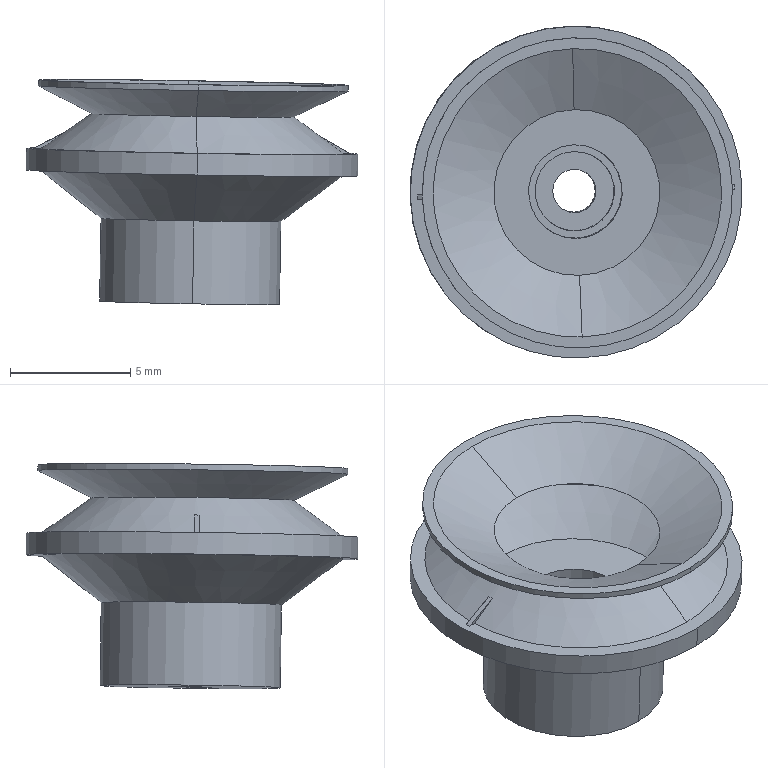Component | SolidWorks | 00-VacuumSuctionCupAssembly-1_08-SoftRubberSuctionCup-28 | 1 solid | 37 faces | box 13.81 x 13.81 x 9.37 mm | volume 326 mm3 | plane 13 | cylinder 12 | cone 12 | commonest cylinder face diameters 1.8 x2 3.9 x2 3.3 x2 7.5 x2 12.9 x2 13.8 x2
STEP:
#1=COLOUR_RGB('',0.7922,0.8196,0.9333);
#2=FILL_AREA_STYLE_COLOUR('',#1);
#3=FILL_AREA_STYLE('',(#2));
#4=SURFACE_STYLE_FILL_AREA(#3);
#5=SURFACE_SIDE_STYLE('',(#4));
#6=SURFACE_STYLE_USAGE(.BOTH.,#5);
#7=PRESENTATION_STYLE_ASSIGNMENT((#6));
#8=CARTESIAN_POINT('',(1.624,5.222,2.221));
#9=VERTEX_POINT('',#8);
#10=CARTESIAN_POINT('',(1.622,5.292,2.222));
#11=VERTEX_POINT('',#10);
#12=CARTESIAN_POINT('',(1.623,5.257,2.222));
#13=DIRECTION('',(0.01745,-0.01259,0.9998));
#14=DIRECTION('',(0.03309,-0.9994,-0.01316));
#15=AXIS2_PLACEMENT_3D('',#12,#13,#14);
#16=CIRCLE('',#15,0.03543);
#17=EDGE_CURVE('',#9,#11,#16,.T.);
#18=ORIENTED_EDGE('',*,*,#17,.F.);
#19=CARTESIAN_POINT('',(1.625,5.221,2.304));
#20=VERTEX_POINT('',#19);
#21=CARTESIAN_POINT('',(1.622,5.223,2.127));
#22=DIRECTION('',(0.01745,-0.01259,0.9998));
#23=VECTOR('',#22,39.37);
#24=LINE('',#21,#23);
#25=EDGE_CURVE('',#9,#20,#24,.T.);
#26=ORIENTED_EDGE('',*,*,#25,.T.);
#27=CARTESIAN_POINT('',(1.623,5.291,2.305));
#28=VERTEX_POINT('',#27);
#29=CARTESIAN_POINT('',(1.624,5.256,2.305));
#30=DIRECTION('',(-0.01745,0.01259,-0.9998));
#31=DIRECTION('',(0.03309,-0.9994,-0.01316));
#32=AXIS2_PLACEMENT_3D('',#29,#30,#31);
#33=CIRCLE('',#32,0.03543);
#34=EDGE_CURVE('',#28,#20,#33,.T.);
#35=ORIENTED_EDGE('',*,*,#34,.F.);
#36=CARTESIAN_POINT('',(1.62,5.294,2.128));
#37=DIRECTION('',(0.01745,-0.01259,0.9998));
#38=VECTOR('',#37,39.37);
#39=LINE('',#36,#38);
#40=EDGE_CURVE('',#11,#28,#39,.T.);
#41=ORIENTED_EDGE('',*,*,#40,.F.);
#42=EDGE_LOOP('',(#18,#26,#35,#41));
#43=FACE_OUTER_BOUND('',#42,.T.);
#44=CARTESIAN_POINT('',(1.621,5.258,2.127));
#45=DIRECTION('',(0.01745,-0.01259,0.9998));
#46=DIRECTION('',(-0.03309,0.9994,0.01316));
#47=AXIS2_PLACEMENT_3D('',#44,#45,#46);
#48=CYLINDRICAL_SURFACE('',#47,0.03543);
#49=ADVANCED_FACE('',(#43),#48,.F.);
#50=CARTESIAN_POINT('',(1.624,5.389,2.531));
#51=VERTEX_POINT('',#50);
#52=CARTESIAN_POINT('',(1.633,5.117,2.527));
#53=VERTEX_POINT('',#52);
#54=CARTESIAN_POINT('',(1.628,5.253,2.529));
#55=DIRECTION('',(-0.01745,0.01259,-0.9998));
#56=DIRECTION('',(0.03309,-0.9994,-0.01316));
#57=AXIS2_PLACEMENT_3D('',#54,#55,#56);
#58=CIRCLE('',#57,0.1358);
#59=EDGE_CURVE('',#51,#53,#58,.T.);
#60=ORIENTED_EDGE('',*,*,#59,.F.);
#61=CARTESIAN_POINT('',(1.619,5.492,2.459));
#62=VERTEX_POINT('',#61);
#63=CARTESIAN_POINT('',(1.619,5.492,2.459));
#64=DIRECTION('',(-0.03707,0.8205,-0.5704));
#65=VECTOR('',#64,39.37);
#66=LINE('',#63,#65);
#67=EDGE_CURVE('',#51,#62,#66,.T.);
#68=ORIENTED_EDGE('',*,*,#67,.T.);
#69=CARTESIAN_POINT('',(1.635,5.016,2.453));
#70=VERTEX_POINT('',#69);
#71=CARTESIAN_POINT('',(1.627,5.254,2.456));
#72=DIRECTION('',(-0.01745,0.01259,-0.9998));
#73=DIRECTION('',(0.03309,-0.9994,-0.01316));
#74=AXIS2_PLACEMENT_3D('',#71,#72,#73);
#75=CIRCLE('',#74,0.2381);
#76=EDGE_CURVE('',#62,#70,#75,.T.);
#77=ORIENTED_EDGE('',*,*,#76,.T.);
#78=CARTESIAN_POINT('',(1.635,5.016,2.453));
#79=DIRECTION('',(0.01679,-0.8059,-0.5918));
#80=VECTOR('',#79,39.37);
#81=LINE('',#78,#80);
#82=EDGE_CURVE('',#53,#70,#81,.T.);
#83=ORIENTED_EDGE('',*,*,#82,.F.);
#84=EDGE_LOOP('',(#60,#68,#77,#83));
#85=FACE_OUTER_BOUND('',#84,.T.);
#86=CARTESIAN_POINT('',(1.627,5.254,2.456));
#87=DIRECTION('',(-0.01745,0.01259,-0.9998));
#88=DIRECTION('',(0.03309,-0.9994,-0.01316));
#89=AXIS2_PLACEMENT_3D('',#86,#87,#88);
#90=CONICAL_SURFACE('',#89,0.2381,0.9505);
#91=ADVANCED_FACE('',(#85),#90,.F.);
#92=CARTESIAN_POINT('',(1.621,5.418,2.401));
#93=VERTEX_POINT('',#92);
#94=CARTESIAN_POINT('',(1.631,5.091,2.397));
#95=VERTEX_POINT('',#94);
#96=CARTESIAN_POINT('',(1.626,5.255,2.399));
#97=DIRECTION('',(-0.01745,0.01259,-0.9998));
#98=DIRECTION('',(0.03309,-0.9994,-0.01316));
#99=AXIS2_PLACEMENT_3D('',#96,#97,#98);
#100=CIRCLE('',#99,0.1636);
#101=EDGE_CURVE('',#93,#95,#100,.T.);
#102=ORIENTED_EDGE('',*,*,#101,.T.);
#103=CARTESIAN_POINT('',(1.631,5.091,2.397));
#104=DIRECTION('',(0.03689,-0.8015,0.5969));
#105=VECTOR('',#104,39.37);
#106=LINE('',#103,#105);
#107=EDGE_CURVE('',#95,#70,#106,.T.);
#108=ORIENTED_EDGE('',*,*,#107,.T.);
#109=ORIENTED_EDGE('',*,*,#76,.F.);
#110=CARTESIAN_POINT('',(1.621,5.418,2.401));
#111=DIRECTION('',(-0.01569,0.7862,0.6178));
#112=VECTOR('',#111,39.37);
#113=LINE('',#110,#112);
#114=EDGE_CURVE('',#93,#62,#113,.T.);
#115=ORIENTED_EDGE('',*,*,#114,.F.);
#116=EDGE_LOOP('',(#102,#108,#109,#115));
#117=FACE_OUTER_BOUND('',#116,.T.);
#118=CARTESIAN_POINT('',(1.626,5.255,2.399));
#119=DIRECTION('',(0.01745,-0.01259,0.9998));
#120=DIRECTION('',(-0.03309,0.9994,0.01316));
#121=AXIS2_PLACEMENT_3D('',#118,#119,#120);
#122=CONICAL_SURFACE('',#121,0.1636,0.9179);
#123=ADVANCED_FACE('',(#117),#122,.F.);
#124=CARTESIAN_POINT('',(1.623,5.331,2.4));
#125=VERTEX_POINT('',#124);
#126=CARTESIAN_POINT('',(1.629,5.178,2.398));
#127=VERTEX_POINT('',#126);
#128=CARTESIAN_POINT('',(1.626,5.255,2.399));
#129=DIRECTION('',(-0.01745,0.01259,-0.9998));
#130=DIRECTION('',(0.03309,-0.9994,-0.01316));
#131=AXIS2_PLACEMENT_3D('',#128,#129,#130);
#132=CIRCLE('',#131,0.07677);
#133=EDGE_CURVE('',#125,#127,#132,.T.);
#134=ORIENTED_EDGE('',*,*,#133,.F.);
#135=CARTESIAN_POINT('',(1.622,5.332,2.341));
#136=VERTEX_POINT('',#135);
#137=CARTESIAN_POINT('',(1.627,5.329,2.583));
#138=DIRECTION('',(-0.01745,0.01259,-0.9998));
#139=VECTOR('',#138,39.37);
#140=LINE('',#137,#139);
#141=EDGE_CURVE('',#125,#136,#140,.T.);
#142=ORIENTED_EDGE('',*,*,#141,.T.);
#143=CARTESIAN_POINT('',(1.627,5.179,2.339));
#144=VERTEX_POINT('',#143);
#145=CARTESIAN_POINT('',(1.625,5.255,2.34));
#146=DIRECTION('',(-0.01745,0.01259,-0.9998));
#147=DIRECTION('',(0.03309,-0.9994,-0.01316));
#148=AXIS2_PLACEMENT_3D('',#145,#146,#147);
#149=CIRCLE('',#148,0.07677);
#150=EDGE_CURVE('',#136,#144,#149,.T.);
#151=ORIENTED_EDGE('',*,*,#150,.T.);
#152=CARTESIAN_POINT('',(1.632,5.176,2.581));
#153=DIRECTION('',(-0.01745,0.01259,-0.9998));
#154=VECTOR('',#153,39.37);
#155=LINE('',#152,#154);
#156=EDGE_CURVE('',#127,#144,#155,.T.);
#157=ORIENTED_EDGE('',*,*,#156,.F.);
#158=EDGE_LOOP('',(#134,#142,#151,#157));
#159=FACE_OUTER_BOUND('',#158,.T.);
#160=CARTESIAN_POINT('',(1.629,5.252,2.582));
#161=DIRECTION('',(-0.01745,0.01259,-0.9998));
#162=DIRECTION('',(0.03309,-0.9994,-0.01316));
#163=AXIS2_PLACEMENT_3D('',#160,#161,#162);
#164=CYLINDRICAL_SURFACE('',#163,0.07677);
#165=ADVANCED_FACE('',(#159),#164,.F.);
#166=CARTESIAN_POINT('',(1.623,5.32,2.341));
#167=VERTEX_POINT('',#166);
#168=CARTESIAN_POINT('',(1.627,5.191,2.339));
#169=VERTEX_POINT('',#168);
#170=CARTESIAN_POINT('',(1.625,5.255,2.34));
#171=DIRECTION('',(-0.01745,0.01259,-0.9998));
#172=DIRECTION('',(0.03309,-0.9994,-0.01316));
#173=AXIS2_PLACEMENT_3D('',#170,#171,#172);
#174=CIRCLE('',#173,0.06496);
#175=EDGE_CURVE('',#167,#169,#174,.T.);
#176=ORIENTED_EDGE('',*,*,#175,.F.);
#177=CARTESIAN_POINT('',(1.622,5.321,2.305));
#178=VERTEX_POINT('',#177);
#179=CARTESIAN_POINT('',(1.627,5.317,2.583));
#180=DIRECTION('',(-0.01745,0.01259,-0.9998));
#181=VECTOR('',#180,39.37);
#182=LINE('',#179,#181);
#183=EDGE_CURVE('',#167,#178,#182,.T.);
#184=ORIENTED_EDGE('',*,*,#183,.T.);
#185=CARTESIAN_POINT('',(1.626,5.191,2.304));
#186=VERTEX_POINT('',#185);
#187=CARTESIAN_POINT('',(1.624,5.256,2.305));
#188=DIRECTION('',(-0.01745,0.01259,-0.9998));
#189=DIRECTION('',(0.03309,-0.9994,-0.01316));
#190=AXIS2_PLACEMENT_3D('',#187,#188,#189);
#191=CIRCLE('',#190,0.06496);
#192=EDGE_CURVE('',#178,#186,#191,.T.);
#193=ORIENTED_EDGE('',*,*,#192,.T.);
#194=CARTESIAN_POINT('',(1.631,5.188,2.581));
#195=DIRECTION('',(-0.01745,0.01259,-0.9998));
#196=VECTOR('',#195,39.37);
#197=LINE('',#194,#196);
#198=EDGE_CURVE('',#169,#186,#197,.T.);
#199=ORIENTED_EDGE('',*,*,#198,.F.);
#200=EDGE_LOOP('',(#176,#184,#193,#199));
#201=FACE_OUTER_BOUND('',#200,.T.);
#202=CARTESIAN_POINT('',(1.629,5.252,2.582));
#203=DIRECTION('',(-0.01745,0.01259,-0.9998));
#204=DIRECTION('',(0.03309,-0.9994,-0.01316));
#205=AXIS2_PLACEMENT_3D('',#202,#203,#204);
#206=CYLINDRICAL_SURFACE('',#205,0.06496);
#207=ADVANCED_FACE('',(#201),#206,.F.);
#208=ORIENTED_EDGE('',*,*,#59,.T.);
#209=CARTESIAN_POINT('',(1.637,5.016,2.579));
#210=VERTEX_POINT('',#209);
#211=CARTESIAN_POINT('',(1.633,5.117,2.527));
#212=DIRECTION('',(0.03741,-0.8891,0.4561));
#213=VECTOR('',#212,39.37);
#214=LINE('',#211,#213);
#215=EDGE_CURVE('',#53,#210,#214,.T.);
#216=ORIENTED_EDGE('',*,*,#215,.T.);
#217=CARTESIAN_POINT('',(1.621,5.489,2.585));
#218=VERTEX_POINT('',#217);
#219=CARTESIAN_POINT('',(1.629,5.252,2.582));
#220=DIRECTION('',(-0.01745,0.01259,-0.9998));
#221=DIRECTION('',(0.03309,-0.9994,-0.01316));
#222=AXIS2_PLACEMENT_3D('',#219,#220,#221);
#223=CIRCLE('',#222,0.2362);
#224=EDGE_CURVE('',#218,#210,#223,.T.);
#225=ORIENTED_EDGE('',*,*,#224,.F.);
#226=CARTESIAN_POINT('',(1.624,5.389,2.531));
#227=DIRECTION('',(-0.02108,0.8773,0.4794));
#228=VECTOR('',#227,39.37);
#229=LINE('',#226,#228);
#230=EDGE_CURVE('',#51,#218,#229,.T.);
#231=ORIENTED_EDGE('',*,*,#230,.F.);
#232=EDGE_LOOP('',(#208,#216,#225,#231));
#233=FACE_OUTER_BOUND('',#232,.T.);
#234=CARTESIAN_POINT('',(1.628,5.253,2.529));
#235=DIRECTION('',(0.01745,-0.01259,0.9998));
#236=DIRECTION('',(-0.03309,0.9994,0.01316));
#237=AXIS2_PLACEMENT_3D('',#234,#235,#236);
#238=CONICAL_SURFACE('',#237,0.1358,1.084);
#239=ADVANCED_FACE('',(#233),#238,.F.);
#240=CARTESIAN_POINT('',(1.628,5.109,2.22));
#241=VERTEX_POINT('',#240);
#242=CARTESIAN_POINT('',(1.618,5.405,2.224));
#243=VERTEX_POINT('',#242);
#244=CARTESIAN_POINT('',(1.623,5.257,2.222));
#245=DIRECTION('',(-0.01745,0.01259,-0.9998));
#246=DIRECTION('',(0.03309,-0.9994,-0.01316));
#247=AXIS2_PLACEMENT_3D('',#244,#245,#246);
#248=CIRCLE('',#247,0.1476);
#249=EDGE_CURVE('',#241,#243,#248,.T.);
#250=ORIENTED_EDGE('',*,*,#249,.F.);
#251=CARTESIAN_POINT('',(1.63,5.108,2.356));
#252=VERTEX_POINT('',#251);
#253=CARTESIAN_POINT('',(1.628,5.109,2.22));
#254=DIRECTION('',(0.01745,-0.01259,0.9998));
#255=VECTOR('',#254,39.37);
#256=LINE('',#253,#255);
#257=EDGE_CURVE('',#241,#252,#256,.T.);
#258=ORIENTED_EDGE('',*,*,#257,.T.);
#259=CARTESIAN_POINT('',(1.62,5.403,2.36));
#260=VERTEX_POINT('',#259);
#261=CARTESIAN_POINT('',(1.625,5.255,2.358));
#262=DIRECTION('',(-0.01745,0.01259,-0.9998));
#263=DIRECTION('',(0.03309,-0.9994,-0.01316));
#264=AXIS2_PLACEMENT_3D('',#261,#262,#263);
#265=CIRCLE('',#264,0.1476);
#266=EDGE_CURVE('',#252,#260,#265,.T.);
#267=ORIENTED_EDGE('',*,*,#266,.T.);
#268=CARTESIAN_POINT('',(1.618,5.405,2.224));
#269=DIRECTION('',(0.01745,-0.01259,0.9998));
#270=VECTOR('',#269,39.37);
#271=LINE('',#268,#270);
#272=EDGE_CURVE('',#243,#260,#271,.T.);
#273=ORIENTED_EDGE('',*,*,#272,.F.);
#274=EDGE_LOOP('',(#250,#258,#267,#273));
#275=FACE_OUTER_BOUND('',#274,.T.);
#276=CARTESIAN_POINT('',(1.623,5.257,2.222));
#277=DIRECTION('',(0.01745,-0.01259,0.9998));
#278=DIRECTION('',(-0.03309,0.9994,0.01316));
#279=AXIS2_PLACEMENT_3D('',#276,#277,#278);
#280=CYLINDRICAL_SURFACE('',#279,0.1476);
#281=ADVANCED_FACE('',(#275),#280,.T.);
#282=CARTESIAN_POINT('',(1.625,5.255,2.358));
#283=DIRECTION('',(-0.01745,0.01259,-0.9998));
#284=DIRECTION('',(0.03309,-0.9994,-0.01316));
#285=AXIS2_PLACEMENT_3D('',#282,#283,#284);
#286=CIRCLE('',#285,0.1476);
#287=EDGE_CURVE('',#260,#252,#286,.T.);
#288=ORIENTED_EDGE('',*,*,#287,.F.);
#289=CARTESIAN_POINT('',(1.618,5.502,2.438));
#290=VERTEX_POINT('',#289);
#291=CARTESIAN_POINT('',(1.618,5.502,2.438));
#292=DIRECTION('',(-0.01569,0.7862,0.6178));
#293=VECTOR('',#292,39.37);
#294=LINE('',#291,#293);
#295=EDGE_CURVE('',#260,#290,#294,.T.);
#296=ORIENTED_EDGE('',*,*,#295,.T.);
#297=CARTESIAN_POINT('',(1.635,5.006,2.431));
#298=VERTEX_POINT('',#297);
#299=CARTESIAN_POINT('',(1.627,5.254,2.434));
#300=DIRECTION('',(-0.01745,0.01259,-0.9998));
#301=DIRECTION('',(0.03309,-0.9994,-0.01316));
#302=AXIS2_PLACEMENT_3D('',#299,#300,#301);
#303=CIRCLE('',#302,0.248);
#304=EDGE_CURVE('',#290,#298,#303,.T.);
#305=ORIENTED_EDGE('',*,*,#304,.T.);
#306=CARTESIAN_POINT('',(1.635,5.006,2.431));
#307=DIRECTION('',(0.03689,-0.8015,0.5969));
#308=VECTOR('',#307,39.37);
#309=LINE('',#306,#308);
#310=EDGE_CURVE('',#252,#298,#309,.T.);
#311=ORIENTED_EDGE('',*,*,#310,.F.);
#312=EDGE_LOOP('',(#288,#296,#305,#311));
#313=FACE_OUTER_BOUND('',#312,.T.);
#314=CARTESIAN_POINT('',(1.627,5.254,2.434));
#315=DIRECTION('',(0.01745,-0.01259,0.9998));
#316=DIRECTION('',(0.03309,-0.9994,-0.01316));
#317=AXIS2_PLACEMENT_3D('',#314,#315,#316);
#318=CONICAL_SURFACE('',#317,0.248,0.9179);
#319=ADVANCED_FACE('',(#313),#318,.T.);
#320=CARTESIAN_POINT('',(1.621,5.506,2.585));
#321=VERTEX_POINT('',#320);
#322=CARTESIAN_POINT('',(1.638,4.999,2.579));
#323=VERTEX_POINT('',#322);
#324=CARTESIAN_POINT('',(1.629,5.252,2.582));
#325=DIRECTION('',(0.01745,-0.01259,0.9998));
#326=DIRECTION('',(-0.03309,0.9994,0.01316));
#327=AXIS2_PLACEMENT_3D('',#324,#325,#326);
#328=CIRCLE('',#327,0.2539);
#329=EDGE_CURVE('',#321,#323,#328,.T.);
#330=ORIENTED_EDGE('',*,*,#329,.F.);
#331=CARTESIAN_POINT('',(1.621,5.506,2.576));
#332=VERTEX_POINT('',#331);
#333=CARTESIAN_POINT('',(1.621,5.506,2.585));
#334=DIRECTION('',(-0.01745,0.01259,-0.9998));
#335=VECTOR('',#334,39.37);
#336=LINE('',#333,#335);
#337=EDGE_CURVE('',#321,#332,#336,.T.);
#338=ORIENTED_EDGE('',*,*,#337,.T.);
#339=CARTESIAN_POINT('',(1.637,4.999,2.569));
#340=VERTEX_POINT('',#339);
#341=CARTESIAN_POINT('',(1.629,5.253,2.573));
#342=DIRECTION('',(0.01745,-0.01259,0.9998));
#343=DIRECTION('',(-0.03309,0.9994,0.01316));
#344=AXIS2_PLACEMENT_3D('',#341,#342,#343);
#345=CIRCLE('',#344,0.2539);
#346=EDGE_CURVE('',#332,#340,#345,.T.);
#347=ORIENTED_EDGE('',*,*,#346,.T.);
#348=CARTESIAN_POINT('',(1.638,4.999,2.579));
#349=DIRECTION('',(-0.01745,0.01259,-0.9998));
#350=VECTOR('',#349,39.37);
#351=LINE('',#348,#350);
#352=EDGE_CURVE('',#323,#340,#351,.T.);
#353=ORIENTED_EDGE('',*,*,#352,.F.);
#354=EDGE_LOOP('',(#330,#338,#347,#353));
#355=FACE_OUTER_BOUND('',#354,.T.);
#356=CARTESIAN_POINT('',(1.629,5.252,2.582));
#357=DIRECTION('',(-0.01745,0.01259,-0.9998));
#358=DIRECTION('',(0.03309,-0.9994,-0.01316));
#359=AXIS2_PLACEMENT_3D('',#356,#357,#358);
#360=CYLINDRICAL_SURFACE('',#359,0.2539);
#361=ADVANCED_FACE('',(#355),#360,.T.);
#362=CARTESIAN_POINT('',(1.623,5.418,2.531));
#363=VERTEX_POINT('',#362);
#364=CARTESIAN_POINT('',(1.634,5.088,2.527));
#365=VERTEX_POINT('',#364);
#366=CARTESIAN_POINT('',(1.628,5.253,2.529));
#367=DIRECTION('',(0.01745,-0.01259,0.9998));
#368=DIRECTION('',(-0.03309,0.9994,0.01316));
#369=AXIS2_PLACEMENT_3D('',#366,#367,#368);
#370=CIRCLE('',#369,0.1654);
#371=EDGE_CURVE('',#363,#365,#370,.T.);
#372=ORIENTED_EDGE('',*,*,#371,.T.);
#373=CARTESIAN_POINT('',(1.634,5.088,2.527));
#374=DIRECTION('',(0.0374,-0.9018,0.4305));
#375=VECTOR('',#374,39.37);
#376=LINE('',#373,#375);
#377=EDGE_CURVE('',#365,#340,#376,.T.);
#378=ORIENTED_EDGE('',*,*,#377,.T.);
#379=ORIENTED_EDGE('',*,*,#346,.F.);
#380=CARTESIAN_POINT('',(1.623,5.418,2.531));
#381=DIRECTION('',(-0.02196,0.8907,0.4541));
#382=VECTOR('',#381,39.37);
#383=LINE('',#380,#382);
#384=EDGE_CURVE('',#363,#332,#383,.T.);
#385=ORIENTED_EDGE('',*,*,#384,.F.);
#386=EDGE_LOOP('',(#372,#378,#379,#385));
#387=FACE_OUTER_BOUND('',#386,.T.);
#388=CARTESIAN_POINT('',(1.628,5.253,2.529));
#389=DIRECTION('',(0.01745,-0.01259,0.9998));
#390=DIRECTION('',(-0.03309,0.9994,0.01316));
#391=AXIS2_PLACEMENT_3D('',#388,#389,#390);
#392=CONICAL_SURFACE('',#391,0.1654,1.112);
#393=ADVANCED_FACE('',(#387),#392,.T.);
#394=CARTESIAN_POINT('',(1.628,5.253,2.529));
#395=DIRECTION('',(0.01745,-0.01259,0.9998));
#396=DIRECTION('',(-0.03309,0.9994,0.01316));
#397=AXIS2_PLACEMENT_3D('',#394,#395,#396);
#398=CIRCLE('',#397,0.1654);
#399=EDGE_CURVE('',#365,#363,#398,.T.);
#400=ORIENTED_EDGE('',*,*,#399,.F.);
#401=CARTESIAN_POINT('',(1.635,5.006,2.467));
#402=VERTEX_POINT('',#401);
#403=CARTESIAN_POINT('',(1.635,5.006,2.467));
#404=DIRECTION('',(0.01679,-0.8059,-0.5918));
#405=VECTOR('',#404,39.37);
#406=LINE('',#403,#405);
#407=EDGE_CURVE('',#365,#402,#406,.T.);
#408=ORIENTED_EDGE('',*,*,#407,.T.);
#409=CARTESIAN_POINT('',(1.875,5.258,2.466));
#410=VERTEX_POINT('',#409);
#411=CARTESIAN_POINT('',(1.627,5.254,2.47));
#412=DIRECTION('',(0.01745,-0.01259,0.9998));
#413=DIRECTION('',(-0.03309,0.9994,0.01316));
#414=AXIS2_PLACEMENT_3D('',#411,#412,#413);
#415=CIRCLE('',#414,0.248);
#416=EDGE_CURVE('',#402,#410,#415,.T.);
#417=ORIENTED_EDGE('',*,*,#416,.T.);
#418=CARTESIAN_POINT('',(1.834,5.256,2.496));
#419=VERTEX_POINT('',#418);
#420=CARTESIAN_POINT('',(1.875,5.258,2.466));
#421=CARTESIAN_POINT('',(1.862,5.258,2.476));
#422=CARTESIAN_POINT('',(1.848,5.257,2.486));
#423=CARTESIAN_POINT('',(1.834,5.256,2.496));
#424=B_SPLINE_CURVE_WITH_KNOTS('',3,(#420,#421,#422,#423),.UNSPECIFIED.,.F.,.F.,(4,4),(0.0000001,0.001295),.UNSPECIFIED.);
#425=EDGE_CURVE('',#410,#419,#424,.T.);
#426=ORIENTED_EDGE('',*,*,#425,.T.);
#427=CARTESIAN_POINT('',(1.834,5.264,2.496));
#428=VERTEX_POINT('',#427);
#429=CARTESIAN_POINT('',(1.834,5.256,2.496));
#430=CARTESIAN_POINT('',(1.834,5.259,2.496));
#431=CARTESIAN_POINT('',(1.834,5.262,2.496));
#432=CARTESIAN_POINT('',(1.834,5.264,2.496));
#433=(BOUNDED_CURVE()B_SPLINE_CURVE(3,(#429,#430,#431,#432),.UNSPECIFIED.,.F.,.F.)B_SPLINE_CURVE_WITH_KNOTS((4,4),(6.227,6.339),.UNSPECIFIED.)CURVE()GEOMETRIC_REPRESENTATION_ITEM()RATIONAL_B_SPLINE_CURVE((1.,0.999,0.999,1.))REPRESENTATION_ITEM(''));
#434=EDGE_CURVE('',#419,#428,#433,.T.);
#435=ORIENTED_EDGE('',*,*,#434,.T.);
#436=CARTESIAN_POINT('',(1.875,5.266,2.466));
#437=VERTEX_POINT('',#436);
#438=CARTESIAN_POINT('',(1.875,5.266,2.466));
#439=CARTESIAN_POINT('',(1.861,5.266,2.476));
#440=CARTESIAN_POINT('',(1.848,5.265,2.486));
#441=CARTESIAN_POINT('',(1.834,5.264,2.496));
#442=B_SPLINE_CURVE_WITH_KNOTS('',3,(#438,#439,#440,#441),.UNSPECIFIED.,.F.,.F.,(4,4),(0.0000001,0.001295),.UNSPECIFIED.);
#443=EDGE_CURVE('',#437,#428,#442,.T.);
#444=ORIENTED_EDGE('',*,*,#443,.F.);
#445=CARTESIAN_POINT('',(1.619,5.502,2.473));
#446=VERTEX_POINT('',#445);
#447=CARTESIAN_POINT('',(1.627,5.254,2.47));
#448=DIRECTION('',(0.01745,-0.01259,0.9998));
#449=DIRECTION('',(-0.03309,0.9994,0.01316));
#450=AXIS2_PLACEMENT_3D('',#447,#448,#449);
#451=CIRCLE('',#450,0.248);
#452=EDGE_CURVE('',#437,#446,#451,.T.);
#453=ORIENTED_EDGE('',*,*,#452,.T.);
#454=CARTESIAN_POINT('',(1.619,5.502,2.473));
#455=DIRECTION('',(-0.03707,0.8205,-0.5704));
#456=VECTOR('',#455,39.37);
#457=LINE('',#454,#456);
#458=EDGE_CURVE('',#363,#446,#457,.T.);
#459=ORIENTED_EDGE('',*,*,#458,.F.);
#460=EDGE_LOOP('',(#400,#408,#417,#426,#435,#444,#453,#459));
#461=FACE_OUTER_BOUND('',#460,.T.);
#462=CARTESIAN_POINT('',(1.627,5.254,2.47));
#463=DIRECTION('',(-0.01745,0.01259,-0.9998));
#464=DIRECTION('',(-0.03309,0.9994,0.01316));
#465=AXIS2_PLACEMENT_3D('',#462,#463,#464);
#466=CONICAL_SURFACE('',#465,0.248,0.9505);
#467=ADVANCED_FACE('',(#461),#466,.T.);
#468=CARTESIAN_POINT('',(1.618,5.526,2.438));
#469=VERTEX_POINT('',#468);
#470=CARTESIAN_POINT('',(1.636,4.983,2.431));
#471=VERTEX_POINT('',#470);
#472=CARTESIAN_POINT('',(1.627,5.254,2.434));
#473=DIRECTION('',(0.01745,-0.01259,0.9998));
#474=DIRECTION('',(-0.03309,0.9994,0.01316));
#475=AXIS2_PLACEMENT_3D('',#472,#473,#474);
#476=CIRCLE('',#475,0.2717);
#477=EDGE_CURVE('',#469,#471,#476,.T.);
#478=ORIENTED_EDGE('',*,*,#477,.T.);
#479=CARTESIAN_POINT('',(1.636,4.982,2.466));
#480=VERTEX_POINT('',#479);
#481=CARTESIAN_POINT('',(1.636,4.983,2.431));
#482=DIRECTION('',(0.01745,-0.01259,0.9998));
#483=VECTOR('',#482,39.37);
#484=LINE('',#481,#483);
#485=EDGE_CURVE('',#471,#480,#484,.T.);
#486=ORIENTED_EDGE('',*,*,#485,.T.);
#487=CARTESIAN_POINT('',(1.618,5.525,2.473));
#488=VERTEX_POINT('',#487);
#489=CARTESIAN_POINT('',(1.627,5.254,2.47));
#490=DIRECTION('',(0.01745,-0.01259,0.9998));
#491=DIRECTION('',(-0.03309,0.9994,0.01316));
#492=AXIS2_PLACEMENT_3D('',#489,#490,#491);
#493=CIRCLE('',#492,0.2717);
#494=EDGE_CURVE('',#488,#480,#493,.T.);
#495=ORIENTED_EDGE('',*,*,#494,.F.);
#496=CARTESIAN_POINT('',(1.618,5.526,2.438));
#497=DIRECTION('',(0.01745,-0.01259,0.9998));
#498=VECTOR('',#497,39.37);
#499=LINE('',#496,#498);
#500=EDGE_CURVE('',#469,#488,#499,.T.);
#501=ORIENTED_EDGE('',*,*,#500,.F.);
#502=EDGE_LOOP('',(#478,#486,#495,#501));
#503=FACE_OUTER_BOUND('',#502,.T.);
#504=CARTESIAN_POINT('',(1.627,5.254,2.434));
#505=DIRECTION('',(0.01745,-0.01259,0.9998));
#506=DIRECTION('',(-0.03309,0.9994,0.01316));
#507=AXIS2_PLACEMENT_3D('',#504,#505,#506);
#508=CYLINDRICAL_SURFACE('',#507,0.2717);
#509=ADVANCED_FACE('',(#503),#508,.T.);
#510=CARTESIAN_POINT('',(1.627,5.254,2.434));
#511=DIRECTION('',(-0.01745,0.01259,-0.9998));
#512=DIRECTION('',(0.03309,-0.9994,-0.01316));
#513=AXIS2_PLACEMENT_3D('',#510,#511,#512);
#514=CIRCLE('',#513,0.248);
#515=EDGE_CURVE('',#298,#290,#514,.T.);
#516=ORIENTED_EDGE('',*,*,#515,.F.);
#517=ORIENTED_EDGE('',*,*,#304,.F.);
#518=EDGE_LOOP('',(#516,#517));
#519=FACE_BOUND('',#518,.T.);
#520=ORIENTED_EDGE('',*,*,#477,.F.);
#521=CARTESIAN_POINT('',(1.627,5.254,2.434));
#522=DIRECTION('',(0.01745,-0.01259,0.9998));
#523=DIRECTION('',(-0.03309,0.9994,0.01316));
#524=AXIS2_PLACEMENT_3D('',#521,#522,#523);
#525=CIRCLE('',#524,0.2717);
#526=EDGE_CURVE('',#471,#469,#525,.T.);
#527=ORIENTED_EDGE('',*,*,#526,.F.);
#528=EDGE_LOOP('',(#520,#527));
#529=FACE_OUTER_BOUND('',#528,.T.);
#530=CARTESIAN_POINT('',(1.355,5.245,2.439));
#531=DIRECTION('',(-0.01745,0.01259,-0.9998));
#532=DIRECTION('',(0.03309,-0.9994,-0.01316));
#533=AXIS2_PLACEMENT_3D('',#530,#531,#532);
#534=PLANE('',#533);
#535=ADVANCED_FACE('',(#519,#529),#534,.T.);
#536=CARTESIAN_POINT('',(1.887,5.258,2.465));
#537=VERTEX_POINT('',#536);
#538=CARTESIAN_POINT('',(1.627,5.252,2.47));
#539=DIRECTION('',(0.9995,0.02484,-0.01713));
#540=VECTOR('',#539,39.37);
#541=LINE('',#538,#540);
#542=EDGE_CURVE('',#410,#537,#541,.T.);
#543=ORIENTED_EDGE('',*,*,#542,.F.);
#544=ORIENTED_EDGE('',*,*,#416,.F.);
#545=CARTESIAN_POINT('',(1.38,5.242,2.474));
#546=VERTEX_POINT('',#545);
#547=CARTESIAN_POINT('',(1.627,5.254,2.47));
#548=DIRECTION('',(0.01745,-0.01259,0.9998));
#549=DIRECTION('',(-0.03309,0.9994,0.01316));
#550=AXIS2_PLACEMENT_3D('',#547,#548,#549);
#551=CIRCLE('',#550,0.248);
#552=EDGE_CURVE('',#546,#402,#551,.T.);
#553=ORIENTED_EDGE('',*,*,#552,.F.);
#554=CARTESIAN_POINT('',(1.368,5.241,2.474));
#555=VERTEX_POINT('',#554);
#556=CARTESIAN_POINT('',(1.627,5.252,2.47));
#557=DIRECTION('',(-0.999,-0.04179,0.01691));
#558=VECTOR('',#557,39.37);
#559=LINE('',#556,#558);
#560=EDGE_CURVE('',#546,#555,#559,.T.);
#561=ORIENTED_EDGE('',*,*,#560,.T.);
#562=CARTESIAN_POINT('',(1.367,5.249,2.474));
#563=VERTEX_POINT('',#562);
#564=CARTESIAN_POINT('',(1.368,5.245,2.474));
#565=DIRECTION('',(0.03309,-0.9994,-0.01316));
#566=VECTOR('',#565,39.37);
#567=LINE('',#564,#566);
#568=EDGE_CURVE('',#563,#555,#567,.T.);
#569=ORIENTED_EDGE('',*,*,#568,.F.);
#570=CARTESIAN_POINT('',(1.379,5.25,2.474));
#571=VERTEX_POINT('',#570);
#572=CARTESIAN_POINT('',(1.627,5.256,2.47));
#573=DIRECTION('',(-0.9995,-0.02484,0.01713));
#574=VECTOR('',#573,39.37);
#575=LINE('',#572,#574);
#576=EDGE_CURVE('',#571,#563,#575,.T.);
#577=ORIENTED_EDGE('',*,*,#576,.F.);
#578=CARTESIAN_POINT('',(1.627,5.254,2.47));
#579=DIRECTION('',(0.01745,-0.01259,0.9998));
#580=DIRECTION('',(-0.03309,0.9994,0.01316));
#581=AXIS2_PLACEMENT_3D('',#578,#579,#580);
#582=CIRCLE('',#581,0.248);
#583=EDGE_CURVE('',#446,#571,#582,.T.);
#584=ORIENTED_EDGE('',*,*,#583,.F.);
#585=ORIENTED_EDGE('',*,*,#452,.F.);
#586=CARTESIAN_POINT('',(1.887,5.267,2.466));
#587=VERTEX_POINT('',#586);
#588=CARTESIAN_POINT('',(1.627,5.256,2.47));
#589=DIRECTION('',(0.999,0.04179,-0.01691));
#590=VECTOR('',#589,39.37);
#591=LINE('',#588,#590);
#592=EDGE_CURVE('',#437,#587,#591,.T.);
#593=ORIENTED_EDGE('',*,*,#592,.T.);
#594=CARTESIAN_POINT('',(1.887,5.263,2.465));
#595=DIRECTION('',(-0.03309,0.9994,0.01316));
#596=VECTOR('',#595,39.37);
#597=LINE('',#594,#596);
#598=EDGE_CURVE('',#537,#587,#597,.T.);
#599=ORIENTED_EDGE('',*,*,#598,.F.);
#600=EDGE_LOOP('',(#543,#544,#553,#561,#569,#577,#584,#585,#593,#599));
#601=FACE_BOUND('',#600,.T.);
#602=ORIENTED_EDGE('',*,*,#494,.T.);
#603=CARTESIAN_POINT('',(1.627,5.254,2.47));
#604=DIRECTION('',(0.01745,-0.01259,0.9998));
#605=DIRECTION('',(-0.03309,0.9994,0.01316));
#606=AXIS2_PLACEMENT_3D('',#603,#604,#605);
#607=CIRCLE('',#606,0.2717);
#608=EDGE_CURVE('',#480,#488,#607,.T.);
#609=ORIENTED_EDGE('',*,*,#608,.T.);
#610=EDGE_LOOP('',(#602,#609));
#611=FACE_OUTER_BOUND('',#610,.T.);
#612=CARTESIAN_POINT('',(1.627,5.254,2.47));
#613=DIRECTION('',(0.01745,-0.01259,0.9998));
#614=DIRECTION('',(-0.03309,0.9994,0.01316));
#615=AXIS2_PLACEMENT_3D('',#612,#613,#614);
#616=PLANE('',#615);
#617=ADVANCED_FACE('',(#601,#611),#616,.T.);
#618=ORIENTED_EDGE('',*,*,#485,.F.);
#619=ORIENTED_EDGE('',*,*,#526,.T.);
#620=ORIENTED_EDGE('',*,*,#500,.T.);
#621=ORIENTED_EDGE('',*,*,#608,.F.);
#622=EDGE_LOOP('',(#618,#619,#620,#621));
#623=FACE_OUTER_BOUND('',#622,.T.);
#624=CARTESIAN_POINT('',(1.627,5.254,2.434));
#625=DIRECTION('',(0.01745,-0.01259,0.9998));
#626=DIRECTION('',(-0.03309,0.9994,0.01316));
#627=AXIS2_PLACEMENT_3D('',#624,#625,#626);
#628=CYLINDRICAL_SURFACE('',#627,0.2717);
#629=ADVANCED_FACE('',(#623),#628,.T.);
#630=ORIENTED_EDGE('',*,*,#407,.F.);
#631=ORIENTED_EDGE('',*,*,#371,.F.);
#632=ORIENTED_EDGE('',*,*,#458,.T.);
#633=ORIENTED_EDGE('',*,*,#583,.T.);
#634=CARTESIAN_POINT('',(1.421,5.251,2.503));
#635=VERTEX_POINT('',#634);
#636=CARTESIAN_POINT('',(1.379,5.25,2.474));
#637=CARTESIAN_POINT('',(1.393,5.25,2.484));
#638=CARTESIAN_POINT('',(1.407,5.25,2.493));
#639=CARTESIAN_POINT('',(1.421,5.251,2.503));
#640=B_SPLINE_CURVE_WITH_KNOTS('',3,(#636,#637,#638,#639),.UNSPECIFIED.,.F.,.F.,(4,4),(0.0000001,0.001295),.UNSPECIFIED.);
#641=EDGE_CURVE('',#571,#635,#640,.T.);
#642=ORIENTED_EDGE('',*,*,#641,.T.);
#643=CARTESIAN_POINT('',(1.421,5.243,2.503));
#644=VERTEX_POINT('',#643);
#645=CARTESIAN_POINT('',(1.421,5.251,2.503));
#646=CARTESIAN_POINT('',(1.421,5.248,2.503));
#647=CARTESIAN_POINT('',(1.421,5.245,2.503));
#648=CARTESIAN_POINT('',(1.421,5.243,2.503));
#649=(BOUNDED_CURVE()B_SPLINE_CURVE(3,(#645,#646,#647,#648),.UNSPECIFIED.,.F.,.T.)B_SPLINE_CURVE_WITH_KNOTS((4,4),(6.227,6.339),.UNSPECIFIED.)CURVE()GEOMETRIC_REPRESENTATION_ITEM()RATIONAL_B_SPLINE_CURVE((1.,0.999,0.999,1.))REPRESENTATION_ITEM(''));
#650=EDGE_CURVE('',#635,#644,#649,.T.);
#651=ORIENTED_EDGE('',*,*,#650,.T.);
#652=CARTESIAN_POINT('',(1.38,5.242,2.474));
#653=CARTESIAN_POINT('',(1.394,5.242,2.484));
#654=CARTESIAN_POINT('',(1.407,5.242,2.493));
#655=CARTESIAN_POINT('',(1.421,5.243,2.503));
#656=B_SPLINE_CURVE_WITH_KNOTS('',3,(#652,#653,#654,#655),.UNSPECIFIED.,.F.,.F.,(4,4),(0.0000001,0.001295),.UNSPECIFIED.);
#657=EDGE_CURVE('',#546,#644,#656,.T.);
#658=ORIENTED_EDGE('',*,*,#657,.F.);
#659=ORIENTED_EDGE('',*,*,#552,.T.);
#660=EDGE_LOOP('',(#630,#631,#632,#633,#642,#651,#658,#659));
#661=FACE_OUTER_BOUND('',#660,.T.);
#662=CARTESIAN_POINT('',(1.627,5.254,2.47));
#663=DIRECTION('',(-0.01745,0.01259,-0.9998));
#664=DIRECTION('',(-0.03309,0.9994,0.01316));
#665=AXIS2_PLACEMENT_3D('',#662,#663,#664);
#666=CONICAL_SURFACE('',#665,0.248,0.9505);
#667=ADVANCED_FACE('',(#661),#666,.T.);
#668=ORIENTED_EDGE('',*,*,#377,.F.);
#669=ORIENTED_EDGE('',*,*,#399,.T.);
#670=ORIENTED_EDGE('',*,*,#384,.T.);
#671=CARTESIAN_POINT('',(1.629,5.253,2.573));
#672=DIRECTION('',(0.01745,-0.01259,0.9998));
#673=DIRECTION('',(-0.03309,0.9994,0.01316));
#674=AXIS2_PLACEMENT_3D('',#671,#672,#673);
#675=CIRCLE('',#674,0.2539);
#676=EDGE_CURVE('',#340,#332,#675,.T.);
#677=ORIENTED_EDGE('',*,*,#676,.F.);
#678=EDGE_LOOP('',(#668,#669,#670,#677));
#679=FACE_OUTER_BOUND('',#678,.T.);
#680=CARTESIAN_POINT('',(1.628,5.253,2.529));
#681=DIRECTION('',(0.01745,-0.01259,0.9998));
#682=DIRECTION('',(-0.03309,0.9994,0.01316));
#683=AXIS2_PLACEMENT_3D('',#680,#681,#682);
#684=CONICAL_SURFACE('',#683,0.1654,1.112);
#685=ADVANCED_FACE('',(#679),#684,.T.);
#686=ORIENTED_EDGE('',*,*,#337,.F.);
#687=CARTESIAN_POINT('',(1.629,5.252,2.582));
#688=DIRECTION('',(0.01745,-0.01259,0.9998));
#689=DIRECTION('',(-0.03309,0.9994,0.01316));
#690=AXIS2_PLACEMENT_3D('',#687,#688,#689);
#691=CIRCLE('',#690,0.2539);
#692=EDGE_CURVE('',#323,#321,#691,.T.);
#693=ORIENTED_EDGE('',*,*,#692,.F.);
#694=ORIENTED_EDGE('',*,*,#352,.T.);
#695=ORIENTED_EDGE('',*,*,#676,.T.);
#696=EDGE_LOOP('',(#686,#693,#694,#695));
#697=FACE_OUTER_BOUND('',#696,.T.);
#698=CARTESIAN_POINT('',(1.629,5.252,2.582));
#699=DIRECTION('',(-0.01745,0.01259,-0.9998));
#700=DIRECTION('',(0.03309,-0.9994,-0.01316));
#701=AXIS2_PLACEMENT_3D('',#698,#699,#700);
#702=CYLINDRICAL_SURFACE('',#701,0.2539);
#703=ADVANCED_FACE('',(#697),#702,.T.);
#704=ORIENTED_EDGE('',*,*,#224,.T.);
#705=CARTESIAN_POINT('',(1.629,5.252,2.582));
#706=DIRECTION('',(-0.01745,0.01259,-0.9998));
#707=DIRECTION('',(0.03309,-0.9994,-0.01316));
#708=AXIS2_PLACEMENT_3D('',#705,#706,#707);
#709=CIRCLE('',#708,0.2362);
#710=EDGE_CURVE('',#210,#218,#709,.T.);
#711=ORIENTED_EDGE('',*,*,#710,.T.);
#712=EDGE_LOOP('',(#704,#711));
#713=FACE_BOUND('',#712,.T.);
#714=ORIENTED_EDGE('',*,*,#692,.T.);
#715=ORIENTED_EDGE('',*,*,#329,.T.);
#716=EDGE_LOOP('',(#714,#715));
#717=FACE_OUTER_BOUND('',#716,.T.);
#718=CARTESIAN_POINT('',(1.629,5.252,2.582));
#719=DIRECTION('',(0.01745,-0.01259,0.9998));
#720=DIRECTION('',(-0.03309,0.9994,0.01316));
#721=AXIS2_PLACEMENT_3D('',#718,#719,#720);
#722=PLANE('',#721);
#723=ADVANCED_FACE('',(#713,#717),#722,.T.);
#724=ORIENTED_EDGE('',*,*,#295,.F.);
#725=ORIENTED_EDGE('',*,*,#266,.F.);
#726=ORIENTED_EDGE('',*,*,#310,.T.);
#727=ORIENTED_EDGE('',*,*,#515,.T.);
#728=EDGE_LOOP('',(#724,#725,#726,#727));
#729=FACE_OUTER_BOUND('',#728,.T.);
#730=CARTESIAN_POINT('',(1.627,5.254,2.434));
#731=DIRECTION('',(0.01745,-0.01259,0.9998));
#732=DIRECTION('',(0.03309,-0.9994,-0.01316));
#733=AXIS2_PLACEMENT_3D('',#730,#731,#732);
#734=CONICAL_SURFACE('',#733,0.248,0.9179);
#735=ADVANCED_FACE('',(#729),#734,.T.);
#736=ORIENTED_EDGE('',*,*,#257,.F.);
#737=CARTESIAN_POINT('',(1.623,5.257,2.222));
#738=DIRECTION('',(-0.01745,0.01259,-0.9998));
#739=DIRECTION('',(0.03309,-0.9994,-0.01316));
#740=AXIS2_PLACEMENT_3D('',#737,#738,#739);
#741=CIRCLE('',#740,0.1476);
#742=EDGE_CURVE('',#243,#241,#741,.T.);
#743=ORIENTED_EDGE('',*,*,#742,.F.);
#744=ORIENTED_EDGE('',*,*,#272,.T.);
#745=ORIENTED_EDGE('',*,*,#287,.T.);
#746=EDGE_LOOP('',(#736,#743,#744,#745));
#747=FACE_OUTER_BOUND('',#746,.T.);
#748=CARTESIAN_POINT('',(1.623,5.257,2.222));
#749=DIRECTION('',(0.01745,-0.01259,0.9998));
#750=DIRECTION('',(-0.03309,0.9994,0.01316));
#751=AXIS2_PLACEMENT_3D('',#748,#749,#750);
#752=CYLINDRICAL_SURFACE('',#751,0.1476);
#753=ADVANCED_FACE('',(#747),#752,.T.);
#754=CARTESIAN_POINT('',(1.623,5.257,2.222));
#755=DIRECTION('',(0.01745,-0.01259,0.9998));
#756=DIRECTION('',(0.03309,-0.9994,-0.01316));
#757=AXIS2_PLACEMENT_3D('',#754,#755,#756);
#758=CIRCLE('',#757,0.03543);
#759=EDGE_CURVE('',#11,#9,#758,.T.);
#760=ORIENTED_EDGE('',*,*,#759,.T.);
#761=ORIENTED_EDGE('',*,*,#17,.T.);
#762=EDGE_LOOP('',(#760,#761));
#763=FACE_BOUND('',#762,.T.);
#764=ORIENTED_EDGE('',*,*,#742,.T.);
#765=ORIENTED_EDGE('',*,*,#249,.T.);
#766=EDGE_LOOP('',(#764,#765));
#767=FACE_OUTER_BOUND('',#766,.T.);
#768=CARTESIAN_POINT('',(1.623,5.257,2.222));
#769=DIRECTION('',(-0.01745,0.01259,-0.9998));
#770=DIRECTION('',(0.03309,-0.9994,-0.01316));
#771=AXIS2_PLACEMENT_3D('',#768,#769,#770);
#772=PLANE('',#771);
#773=ADVANCED_FACE('',(#763,#767),#772,.T.);
#774=ORIENTED_EDGE('',*,*,#215,.F.);
#775=CARTESIAN_POINT('',(1.628,5.253,2.529));
#776=DIRECTION('',(-0.01745,0.01259,-0.9998));
#777=DIRECTION('',(0.03309,-0.9994,-0.01316));
#778=AXIS2_PLACEMENT_3D('',#775,#776,#777);
#779=CIRCLE('',#778,0.1358);
#780=EDGE_CURVE('',#53,#51,#779,.T.);
#781=ORIENTED_EDGE('',*,*,#780,.T.);
#782=ORIENTED_EDGE('',*,*,#230,.T.);
#783=ORIENTED_EDGE('',*,*,#710,.F.);
#784=EDGE_LOOP('',(#774,#781,#782,#783));
#785=FACE_OUTER_BOUND('',#784,.T.);
#786=CARTESIAN_POINT('',(1.628,5.253,2.529));
#787=DIRECTION('',(0.01745,-0.01259,0.9998));
#788=DIRECTION('',(-0.03309,0.9994,0.01316));
#789=AXIS2_PLACEMENT_3D('',#786,#787,#788);
#790=CONICAL_SURFACE('',#789,0.1358,1.084);
#791=ADVANCED_FACE('',(#785),#790,.F.);
#792=ORIENTED_EDGE('',*,*,#34,.T.);
#793=CARTESIAN_POINT('',(1.624,5.256,2.305));
#794=DIRECTION('',(-0.01745,0.01259,-0.9998));
#795=DIRECTION('',(0.03309,-0.9994,-0.01316));
#796=AXIS2_PLACEMENT_3D('',#793,#794,#795);
#797=CIRCLE('',#796,0.03543);
#798=EDGE_CURVE('',#20,#28,#797,.T.);
#799=ORIENTED_EDGE('',*,*,#798,.T.);
#800=EDGE_LOOP('',(#792,#799));
#801=FACE_BOUND('',#800,.T.);
#802=CARTESIAN_POINT('',(1.624,5.256,2.305));
#803=DIRECTION('',(-0.01745,0.01259,-0.9998));
#804=DIRECTION('',(0.03309,-0.9994,-0.01316));
#805=AXIS2_PLACEMENT_3D('',#802,#803,#804);
#806=CIRCLE('',#805,0.06496);
#807=EDGE_CURVE('',#186,#178,#806,.T.);
#808=ORIENTED_EDGE('',*,*,#807,.F.);
#809=ORIENTED_EDGE('',*,*,#192,.F.);
#810=EDGE_LOOP('',(#808,#809));
#811=FACE_OUTER_BOUND('',#810,.T.);
#812=CARTESIAN_POINT('',(1.59,5.255,2.305));
#813=DIRECTION('',(-0.01745,0.01259,-0.9998));
#814=DIRECTION('',(0.03309,-0.9994,-0.01316));
#815=AXIS2_PLACEMENT_3D('',#812,#813,#814);
#816=PLANE('',#815);
#817=ADVANCED_FACE('',(#801,#811),#816,.F.);
#818=ORIENTED_EDGE('',*,*,#183,.F.);
#819=CARTESIAN_POINT('',(1.625,5.255,2.34));
#820=DIRECTION('',(-0.01745,0.01259,-0.9998));
#821=DIRECTION('',(0.03309,-0.9994,-0.01316));
#822=AXIS2_PLACEMENT_3D('',#819,#820,#821);
#823=CIRCLE('',#822,0.06496);
#824=EDGE_CURVE('',#169,#167,#823,.T.);
#825=ORIENTED_EDGE('',*,*,#824,.F.);
#826=ORIENTED_EDGE('',*,*,#198,.T.);
#827=ORIENTED_EDGE('',*,*,#807,.T.);
#828=EDGE_LOOP('',(#818,#825,#826,#827));
#829=FACE_OUTER_BOUND('',#828,.T.);
#830=CARTESIAN_POINT('',(1.629,5.252,2.582));
#831=DIRECTION('',(-0.01745,0.01259,-0.9998));
#832=DIRECTION('',(0.03309,-0.9994,-0.01316));
#833=AXIS2_PLACEMENT_3D('',#830,#831,#832);
#834=CYLINDRICAL_SURFACE('',#833,0.06496);
#835=ADVANCED_FACE('',(#829),#834,.F.);
#836=ORIENTED_EDGE('',*,*,#824,.T.);
#837=ORIENTED_EDGE('',*,*,#175,.T.);
#838=EDGE_LOOP('',(#836,#837));
#839=FACE_BOUND('',#838,.T.);
#840=CARTESIAN_POINT('',(1.625,5.255,2.34));
#841=DIRECTION('',(-0.01745,0.01259,-0.9998));
#842=DIRECTION('',(0.03309,-0.9994,-0.01316));
#843=AXIS2_PLACEMENT_3D('',#840,#841,#842);
#844=CIRCLE('',#843,0.07677);
#845=EDGE_CURVE('',#144,#136,#844,.T.);
#846=ORIENTED_EDGE('',*,*,#845,.F.);
#847=ORIENTED_EDGE('',*,*,#150,.F.);
#848=EDGE_LOOP('',(#846,#847));
#849=FACE_OUTER_BOUND('',#848,.T.);
#850=CARTESIAN_POINT('',(1.56,5.253,2.341));
#851=DIRECTION('',(-0.01745,0.01259,-0.9998));
#852=DIRECTION('',(0.03309,-0.9994,-0.01316));
#853=AXIS2_PLACEMENT_3D('',#850,#851,#852);
#854=PLANE('',#853);
#855=ADVANCED_FACE('',(#839,#849),#854,.F.);
#856=ORIENTED_EDGE('',*,*,#141,.F.);
#857=CARTESIAN_POINT('',(1.626,5.255,2.399));
#858=DIRECTION('',(-0.01745,0.01259,-0.9998));
#859=DIRECTION('',(0.03309,-0.9994,-0.01316));
#860=AXIS2_PLACEMENT_3D('',#857,#858,#859);
#861=CIRCLE('',#860,0.07677);
#862=EDGE_CURVE('',#127,#125,#861,.T.);
#863=ORIENTED_EDGE('',*,*,#862,.F.);
#864=ORIENTED_EDGE('',*,*,#156,.T.);
#865=ORIENTED_EDGE('',*,*,#845,.T.);
#866=EDGE_LOOP('',(#856,#863,#864,#865));
#867=FACE_OUTER_BOUND('',#866,.T.);
#868=CARTESIAN_POINT('',(1.629,5.252,2.582));
#869=DIRECTION('',(-0.01745,0.01259,-0.9998));
#870=DIRECTION('',(0.03309,-0.9994,-0.01316));
#871=AXIS2_PLACEMENT_3D('',#868,#869,#870);
#872=CYLINDRICAL_SURFACE('',#871,0.07677);
#873=ADVANCED_FACE('',(#867),#872,.F.);
#874=ORIENTED_EDGE('',*,*,#862,.T.);
#875=ORIENTED_EDGE('',*,*,#133,.T.);
#876=EDGE_LOOP('',(#874,#875));
#877=FACE_BOUND('',#876,.T.);
#878=ORIENTED_EDGE('',*,*,#101,.F.);
#879=CARTESIAN_POINT('',(1.626,5.255,2.399));
#880=DIRECTION('',(-0.01745,0.01259,-0.9998));
#881=DIRECTION('',(0.03309,-0.9994,-0.01316));
#882=AXIS2_PLACEMENT_3D('',#879,#880,#881);
#883=CIRCLE('',#882,0.1636);
#884=EDGE_CURVE('',#95,#93,#883,.T.);
#885=ORIENTED_EDGE('',*,*,#884,.F.);
#886=EDGE_LOOP('',(#878,#885));
#887=FACE_OUTER_BOUND('',#886,.T.);
#888=CARTESIAN_POINT('',(1.549,5.252,2.4));
#889=DIRECTION('',(-0.01745,0.01259,-0.9998));
#890=DIRECTION('',(0.03309,-0.9994,-0.01316));
#891=AXIS2_PLACEMENT_3D('',#888,#889,#890);
#892=PLANE('',#891);
#893=ADVANCED_FACE('',(#877,#887),#892,.F.);
#894=ORIENTED_EDGE('',*,*,#107,.F.);
#895=ORIENTED_EDGE('',*,*,#884,.T.);
#896=ORIENTED_EDGE('',*,*,#114,.T.);
#897=CARTESIAN_POINT('',(1.627,5.254,2.456));
#898=DIRECTION('',(-0.01745,0.01259,-0.9998));
#899=DIRECTION('',(0.03309,-0.9994,-0.01316));
#900=AXIS2_PLACEMENT_3D('',#897,#898,#899);
#901=CIRCLE('',#900,0.2381);
#902=EDGE_CURVE('',#70,#62,#901,.T.);
#903=ORIENTED_EDGE('',*,*,#902,.F.);
#904=EDGE_LOOP('',(#894,#895,#896,#903));
#905=FACE_OUTER_BOUND('',#904,.T.);
#906=CARTESIAN_POINT('',(1.626,5.255,2.399));
#907=DIRECTION('',(0.01745,-0.01259,0.9998));
#908=DIRECTION('',(-0.03309,0.9994,0.01316));
#909=AXIS2_PLACEMENT_3D('',#906,#907,#908);
#910=CONICAL_SURFACE('',#909,0.1636,0.9179);
#911=ADVANCED_FACE('',(#905),#910,.F.);
#912=ORIENTED_EDGE('',*,*,#67,.F.);
#913=ORIENTED_EDGE('',*,*,#780,.F.);
#914=ORIENTED_EDGE('',*,*,#82,.T.);
#915=ORIENTED_EDGE('',*,*,#902,.T.);
#916=EDGE_LOOP('',(#912,#913,#914,#915));
#917=FACE_OUTER_BOUND('',#916,.T.);
#918=CARTESIAN_POINT('',(1.627,5.254,2.456));
#919=DIRECTION('',(-0.01745,0.01259,-0.9998));
#920=DIRECTION('',(0.03309,-0.9994,-0.01316));
#921=AXIS2_PLACEMENT_3D('',#918,#919,#920);
#922=CONICAL_SURFACE('',#921,0.2381,0.9505);
#923=ADVANCED_FACE('',(#917),#922,.F.);
#924=CARTESIAN_POINT('',(1.368,5.241,2.474));
#925=DIRECTION('',(0.882,0.02301,0.4706));
#926=VECTOR('',#925,39.37);
#927=LINE('',#924,#926);
#928=EDGE_CURVE('',#555,#644,#927,.T.);
#929=ORIENTED_EDGE('',*,*,#928,.T.);
#930=ORIENTED_EDGE('',*,*,#650,.F.);
#931=CARTESIAN_POINT('',(1.539,5.254,2.566));
#932=DIRECTION('',(0.882,0.02301,0.4706));
#933=VECTOR('',#932,39.37);
#934=LINE('',#931,#933);
#935=EDGE_CURVE('',#563,#635,#934,.T.);
#936=ORIENTED_EDGE('',*,*,#935,.F.);
#937=ORIENTED_EDGE('',*,*,#568,.T.);
#938=EDGE_LOOP('',(#929,#930,#936,#937));
#939=FACE_OUTER_BOUND('',#938,.T.);
#940=CARTESIAN_POINT('',(1.368,5.245,2.474));
#941=DIRECTION('',(-0.47,-0.02718,0.8822));
#942=DIRECTION('',(0.882,0.02301,0.4706));
#943=AXIS2_PLACEMENT_3D('',#940,#941,#942);
#944=PLANE('',#943);
#945=ADVANCED_FACE('',(#939),#944,.T.);
#946=ORIENTED_EDGE('',*,*,#641,.F.);
#947=ORIENTED_EDGE('',*,*,#576,.T.);
#948=ORIENTED_EDGE('',*,*,#935,.T.);
#949=EDGE_LOOP('',(#946,#947,#948));
#950=FACE_OUTER_BOUND('',#949,.T.);
#951=CARTESIAN_POINT('',(1.539,5.254,2.566));
#952=DIRECTION('',(-0.02489,0.9997,-0.002238));
#953=DIRECTION('',(-0.01694,-0.00266,-0.9999));
#954=AXIS2_PLACEMENT_3D('',#951,#952,#953);
#955=PLANE('',#954);
#956=ADVANCED_FACE('',(#950),#955,.T.);
#957=ORIENTED_EDGE('',*,*,#560,.F.);
#958=ORIENTED_EDGE('',*,*,#657,.T.);
#959=ORIENTED_EDGE('',*,*,#928,.F.);
#960=EDGE_LOOP('',(#957,#958,#959));
#961=FACE_OUTER_BOUND('',#960,.T.);
#962=CARTESIAN_POINT('',(1.539,5.246,2.566));
#963=DIRECTION('',(-0.04129,0.9987,0.02856));
#964=DIRECTION('',(-0.01795,0.02783,-0.9995));
#965=AXIS2_PLACEMENT_3D('',#962,#963,#964);
#966=PLANE('',#965);
#967=ADVANCED_FACE('',(#961),#966,.F.);
#968=CARTESIAN_POINT('',(1.719,5.252,2.563));
#969=DIRECTION('',(-0.8651,-0.03524,0.5004));
#970=VECTOR('',#969,39.37);
#971=LINE('',#968,#970);
#972=EDGE_CURVE('',#537,#419,#971,.T.);
#973=ORIENTED_EDGE('',*,*,#972,.F.);
#974=ORIENTED_EDGE('',*,*,#598,.T.);
#975=CARTESIAN_POINT('',(1.887,5.267,2.466));
#976=DIRECTION('',(-0.8651,-0.03524,0.5004));
#977=VECTOR('',#976,39.37);
#978=LINE('',#975,#977);
#979=EDGE_CURVE('',#587,#428,#978,.T.);
#980=ORIENTED_EDGE('',*,*,#979,.T.);
#981=ORIENTED_EDGE('',*,*,#434,.F.);
#982=EDGE_LOOP('',(#973,#974,#980,#981));
#983=FACE_OUTER_BOUND('',#982,.T.);
#984=CARTESIAN_POINT('',(1.887,5.263,2.465));
#985=DIRECTION('',(0.5006,0.005175,0.8657));
#986=DIRECTION('',(-0.8651,-0.03524,0.5004));
#987=AXIS2_PLACEMENT_3D('',#984,#985,#986);
#988=PLANE('',#987);
#989=ADVANCED_FACE('',(#983),#988,.T.);
#990=ORIENTED_EDGE('',*,*,#425,.F.);
#991=ORIENTED_EDGE('',*,*,#542,.T.);
#992=ORIENTED_EDGE('',*,*,#972,.T.);
#993=EDGE_LOOP('',(#990,#991,#992));
#994=FACE_OUTER_BOUND('',#993,.T.);
#995=CARTESIAN_POINT('',(1.719,5.252,2.563));
#996=DIRECTION('',(0.02435,-0.9993,-0.02827));
#997=DIRECTION('',(0.01795,-0.02783,0.9995));
#998=AXIS2_PLACEMENT_3D('',#995,#996,#997);
#999=PLANE('',#998);
#1000=ADVANCED_FACE('',(#994),#999,.T.);
#1001=ORIENTED_EDGE('',*,*,#592,.F.);
#1002=ORIENTED_EDGE('',*,*,#443,.T.);
#1003=ORIENTED_EDGE('',*,*,#979,.F.);
#1004=EDGE_LOOP('',(#1001,#1002,#1003));
#1005=FACE_OUTER_BOUND('',#1004,.T.);
#1006=CARTESIAN_POINT('',(1.719,5.26,2.563));
#1007=DIRECTION('',(0.04183,-0.9991,0.001949));
#1008=DIRECTION('',(0.01694,0.00266,0.9999));
#1009=AXIS2_PLACEMENT_3D('',#1006,#1007,#1008);
#1010=PLANE('',#1009);
#1011=ADVANCED_FACE('',(#1005),#1010,.F.);
#1012=ORIENTED_EDGE('',*,*,#25,.F.);
#1013=ORIENTED_EDGE('',*,*,#759,.F.);
#1014=ORIENTED_EDGE('',*,*,#40,.T.);
#1015=ORIENTED_EDGE('',*,*,#798,.F.);
#1016=EDGE_LOOP('',(#1012,#1013,#1014,#1015));
#1017=FACE_OUTER_BOUND('',#1016,.T.);
#1018=CARTESIAN_POINT('',(1.621,5.258,2.127));
#1019=DIRECTION('',(0.01745,-0.01259,0.9998));
#1020=DIRECTION('',(-0.03309,0.9994,0.01316));
#1021=AXIS2_PLACEMENT_3D('',#1018,#1019,#1020);
#1022=CYLINDRICAL_SURFACE('',#1021,0.03543);
#1023=ADVANCED_FACE('',(#1017),#1022,.F.);
#1024=CLOSED_SHELL('',(#49,#91,#123,#165,#207,#239,#281,#319,#361,#393,#467,#509,#535,#617,#629,#667,#685,#703,#723,#735,#753,#773,#791,#817,#835,#855,#873,#893,#911,#923,#945,#956,#967,#989,#1000,#1011,#1023));
#1025=MANIFOLD_SOLID_BREP('',#1024);
#1026=STYLED_ITEM('',(#7),#1025);
#1027=(LENGTH_UNIT()NAMED_UNIT(*)SI_UNIT($,.METRE.));
#1028=LENGTH_MEASURE_WITH_UNIT(LENGTH_MEASURE(0.0254),#1027);
#1029=DIMENSIONAL_EXPONENTS(1.,0.,0.,0.,0.,0.,0.);
#1030=(CONVERSION_BASED_UNIT('',#1028)LENGTH_UNIT()NAMED_UNIT(#1029));
#1031=UNCERTAINTY_MEASURE_WITH_UNIT(LENGTH_MEASURE(0.00001),#1030,'','');
#1032=(NAMED_UNIT(*)PLANE_ANGLE_UNIT()SI_UNIT($,.RADIAN.));
#1033=(NAMED_UNIT(*)SI_UNIT($,.STERADIAN.)SOLID_ANGLE_UNIT());
#1034=(GEOMETRIC_REPRESENTATION_CONTEXT(3)GLOBAL_UNCERTAINTY_ASSIGNED_CONTEXT((#1031))GLOBAL_UNIT_ASSIGNED_CONTEXT((#1030,#1032,#1033))REPRESENTATION_CONTEXT('',''));
#1035=MECHANICAL_DESIGN_GEOMETRIC_PRESENTATION_REPRESENTATION('',(#1026),#1034);
#1036=PRESENTATION_LAYER_ASSIGNMENT('','',(#1026));
#1037=CARTESIAN_POINT('',(0.,0.,0.));
#1038=DIRECTION('',(0.,0.,1.));
#1039=DIRECTION('',(1.,0.,0.));
#1040=AXIS2_PLACEMENT_3D('',#1037,#1038,#1039);
#1041=(LENGTH_UNIT()NAMED_UNIT(*)SI_UNIT($,.METRE.));
#1042=LENGTH_MEASURE_WITH_UNIT(LENGTH_MEASURE(0.0254),#1041);
#1043=DIMENSIONAL_EXPONENTS(1.,0.,0.,0.,0.,0.,0.);
#1044=(CONVERSION_BASED_UNIT('',#1042)LENGTH_UNIT()NAMED_UNIT(#1043));
#1045=UNCERTAINTY_MEASURE_WITH_UNIT(LENGTH_MEASURE(0.00001),#1044,'','');
#1046=(NAMED_UNIT(*)PLANE_ANGLE_UNIT()SI_UNIT($,.RADIAN.));
#1047=(NAMED_UNIT(*)SI_UNIT($,.STERADIAN.)SOLID_ANGLE_UNIT());
#1048=(GEOMETRIC_REPRESENTATION_CONTEXT(3)GLOBAL_UNCERTAINTY_ASSIGNED_CONTEXT((#1045))GLOBAL_UNIT_ASSIGNED_CONTEXT((#1044,#1046,#1047))REPRESENTATION_CONTEXT('',''));
#1049=ADVANCED_BREP_SHAPE_REPRESENTATION('',(#1025,#1040),#1048);